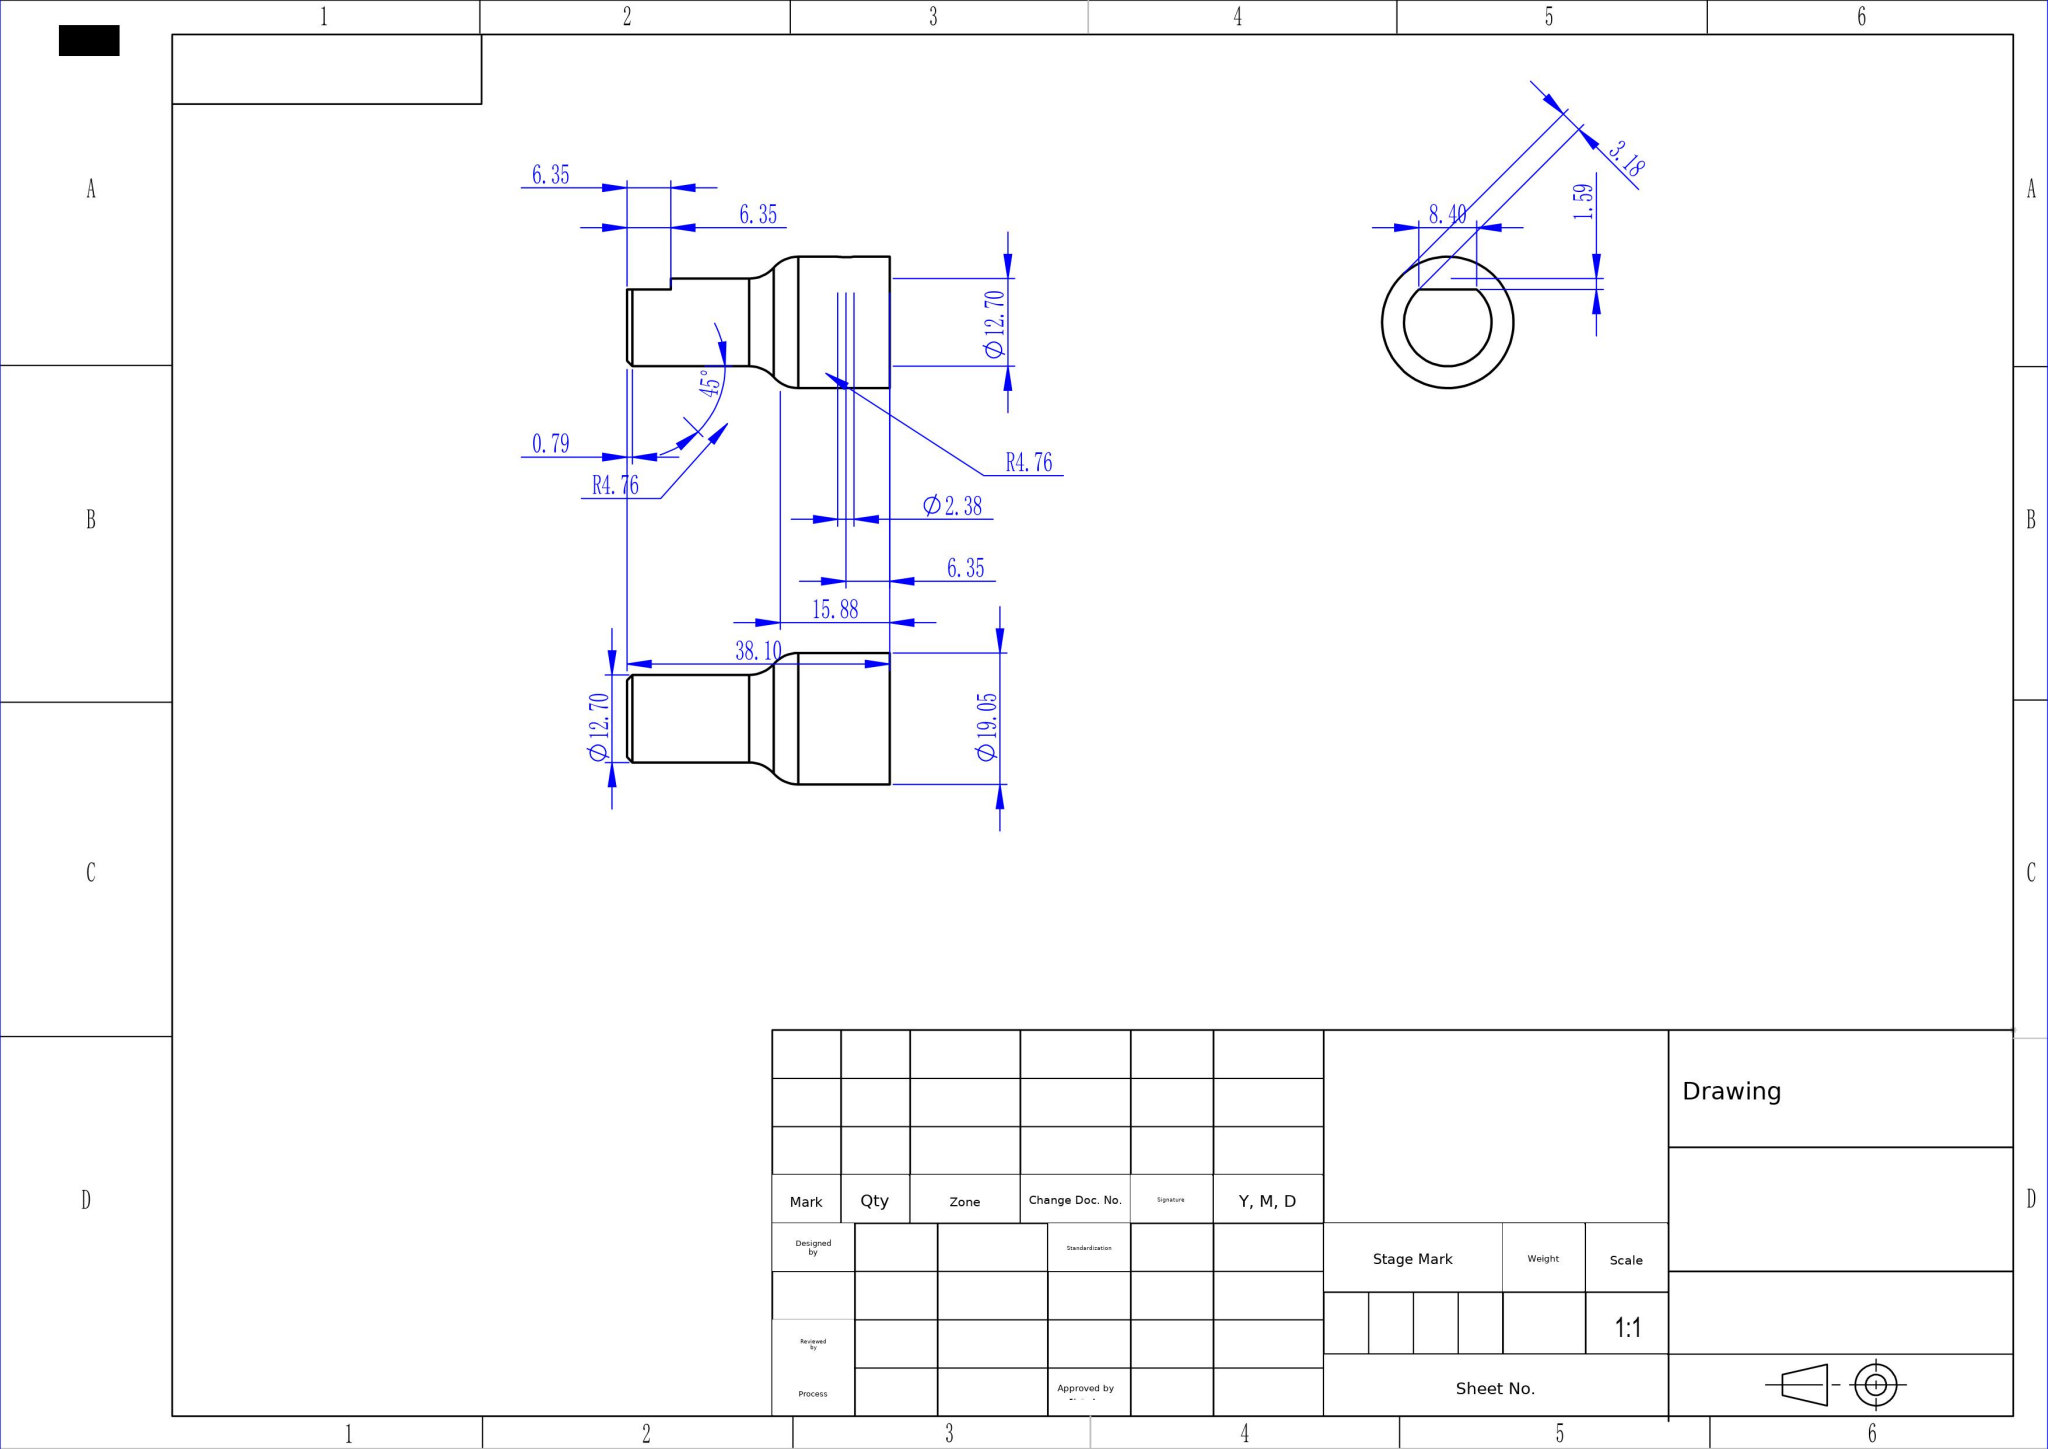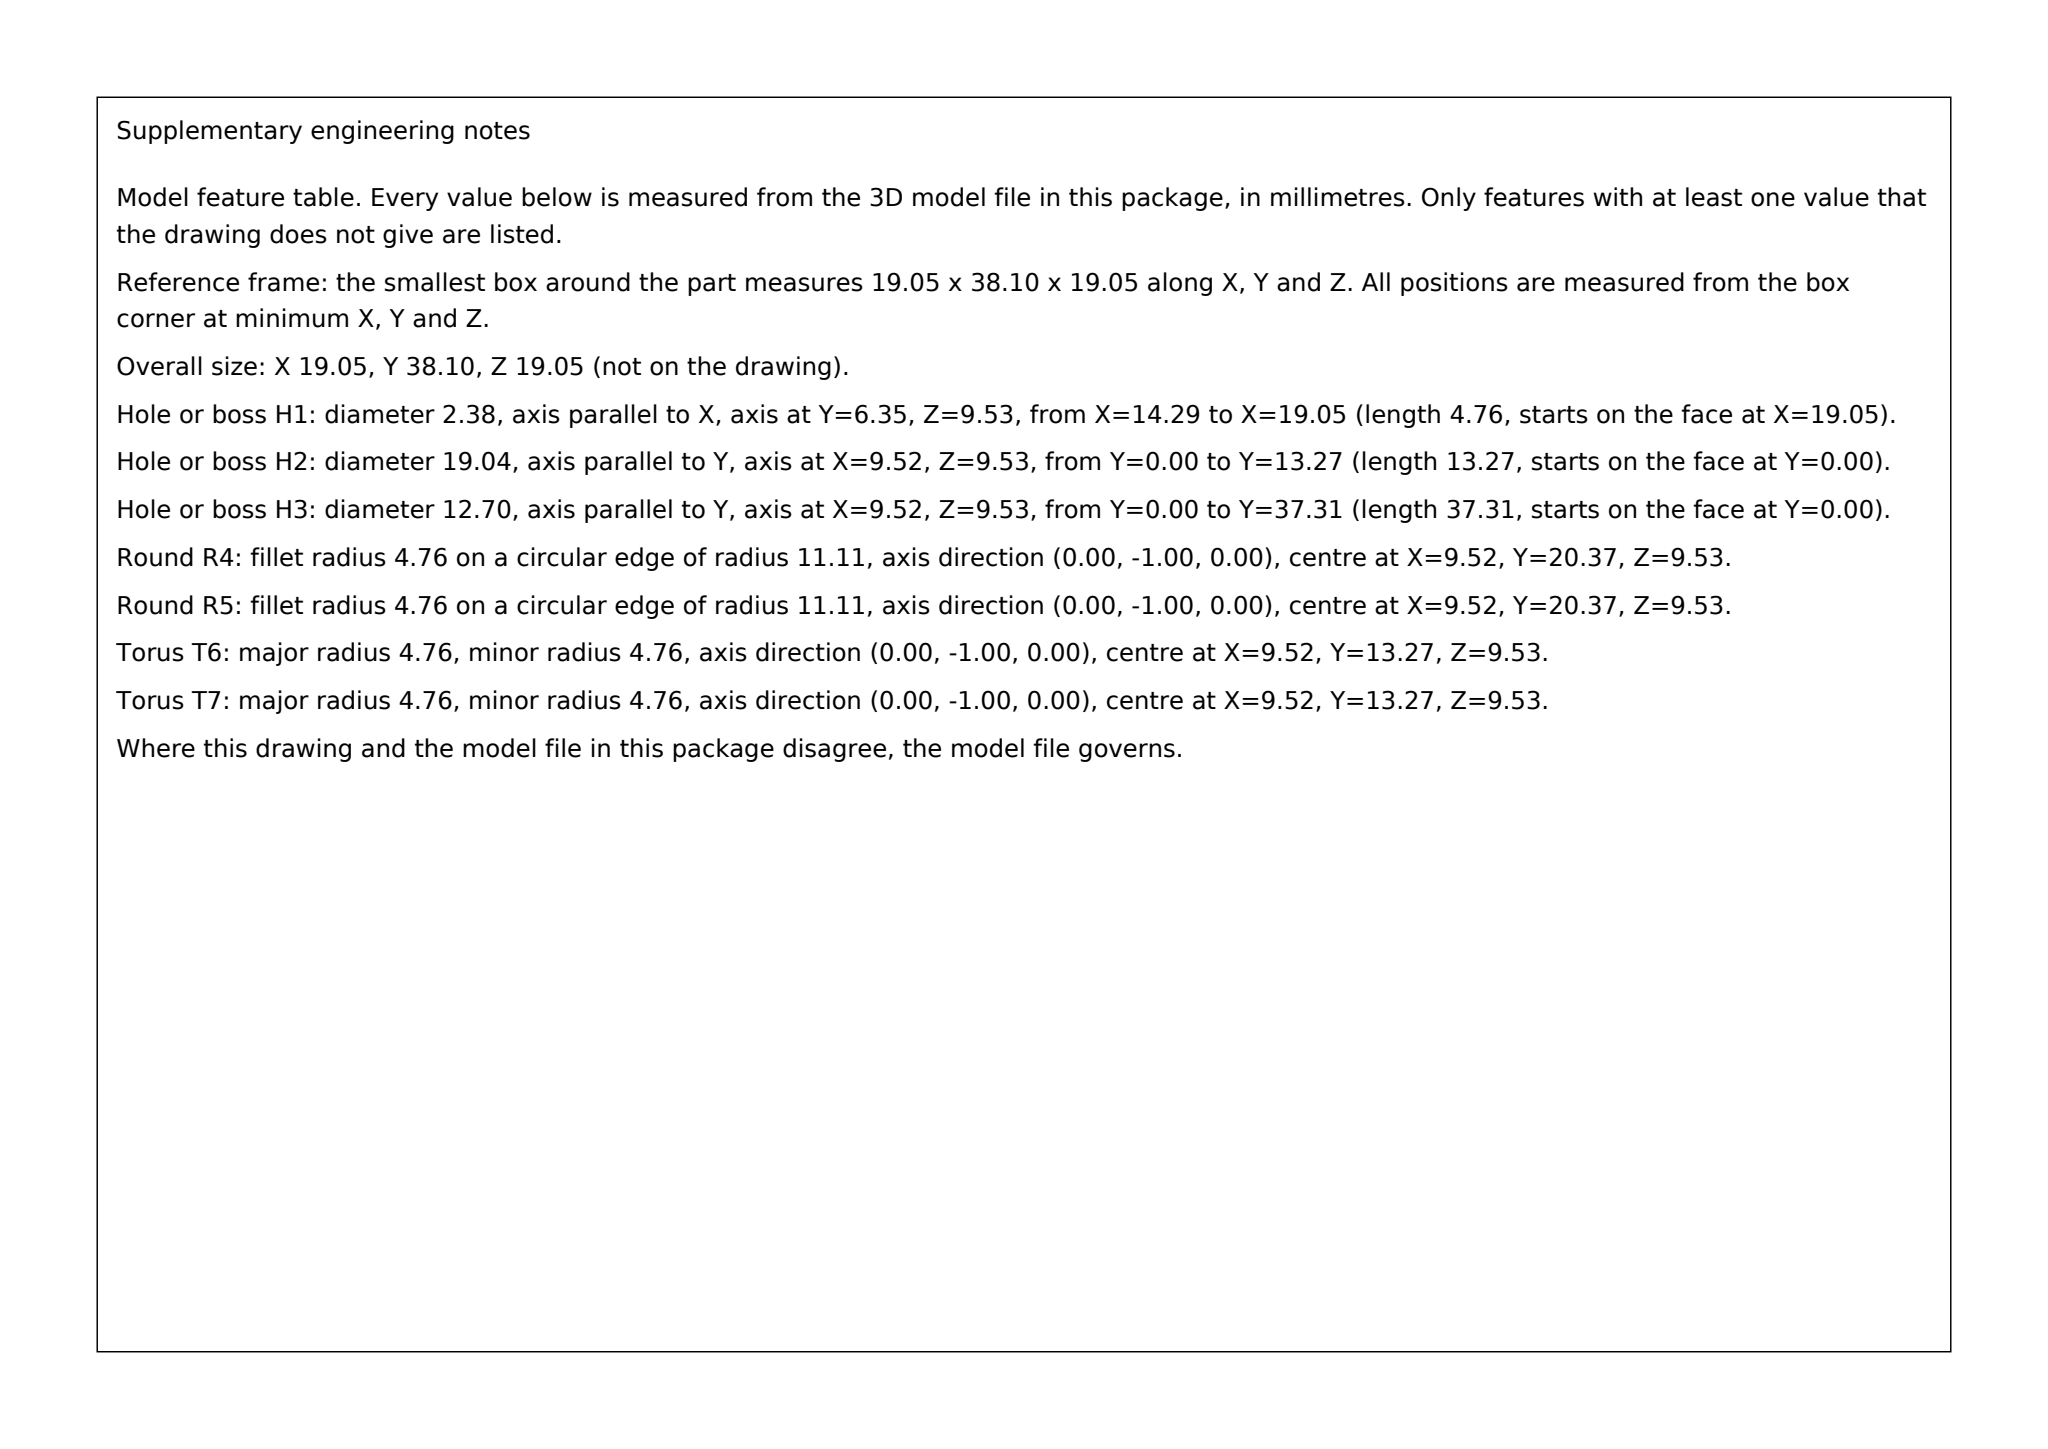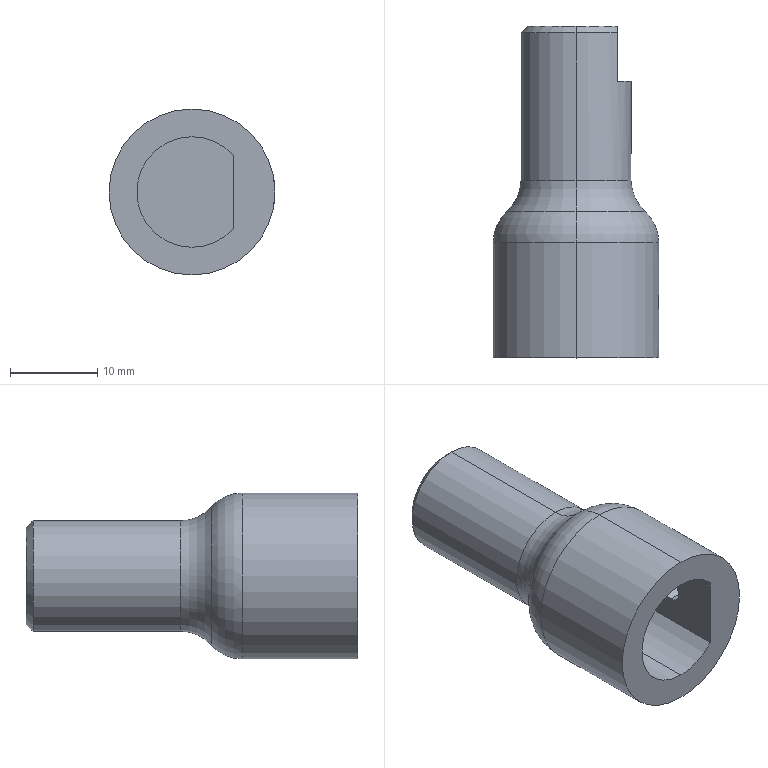Part | SolidWorks | drawing in inches | 1 solid | 22 faces | box 19.05 x 38.1 x 19.05 mm | volume 5883 mm3 | cylinder 9 | plane 6 | torus 4 | cone 3 | commonest cylinder face diameters 12.7 x5 2.381 x2 19.05 x2
STEP:
#1=CARTESIAN_POINT('',(0.,1.5,0.2187));
#2=VERTEX_POINT('',#1);
#3=CARTESIAN_POINT('',(0.1875,1.5,0.1127));
#4=VERTEX_POINT('',#3);
#5=CARTESIAN_POINT('',(0.,1.5,0.));
#6=DIRECTION('',(0.,1.,0.));
#7=DIRECTION('',(0.,0.,1.));
#8=AXIS2_PLACEMENT_3D('',#5,#6,#7);
#9=CIRCLE('',#8,0.2187);
#10=EDGE_CURVE('',#2,#4,#9,.T.);
#11=ORIENTED_EDGE('',*,*,#10,.F.);
#12=CARTESIAN_POINT('',(0.,1.469,0.25));
#13=VERTEX_POINT('',#12);
#14=CARTESIAN_POINT('',(0.,1.5,0.2187));
#15=DIRECTION('',(0.,-0.7071,0.7071));
#16=VECTOR('',#15,39.37);
#17=LINE('',#14,#16);
#18=EDGE_CURVE('',#2,#13,#17,.T.);
#19=ORIENTED_EDGE('',*,*,#18,.T.);
#20=CARTESIAN_POINT('',(0.1875,1.469,0.1654));
#21=VERTEX_POINT('',#20);
#22=CARTESIAN_POINT('',(0.,1.469,0.));
#23=DIRECTION('',(0.,-1.,0.));
#24=DIRECTION('',(0.,0.,1.));
#25=AXIS2_PLACEMENT_3D('',#22,#23,#24);
#26=CIRCLE('',#25,0.25);
#27=EDGE_CURVE('',#21,#13,#26,.T.);
#28=ORIENTED_EDGE('',*,*,#27,.F.);
#29=CARTESIAN_POINT('',(0.1875,1.5,0.1127));
#30=CARTESIAN_POINT('',(0.1875,1.491,0.1309));
#31=CARTESIAN_POINT('',(0.1875,1.48,0.1483));
#32=CARTESIAN_POINT('',(0.1875,1.469,0.1654));
#33=B_SPLINE_CURVE_WITH_KNOTS('',3,(#29,#30,#31,#32),.UNSPECIFIED.,.F.,.F.,(4,4),(0.,0.001556),.UNSPECIFIED.);
#34=EDGE_CURVE('',#4,#21,#33,.T.);
#35=ORIENTED_EDGE('',*,*,#34,.F.);
#36=EDGE_LOOP('',(#11,#19,#28,#35));
#37=FACE_OUTER_BOUND('',#36,.T.);
#38=CARTESIAN_POINT('',(0.,1.5,0.));
#39=DIRECTION('',(0.,-1.,0.));
#40=DIRECTION('',(0.,0.,-1.));
#41=AXIS2_PLACEMENT_3D('',#38,#39,#40);
#42=CONICAL_SURFACE('',#41,0.2187,0.7854);
#43=ADVANCED_FACE('',(#37),#42,.T.);
#44=ORIENTED_EDGE('',*,*,#18,.F.);
#45=CARTESIAN_POINT('',(0.,1.5,-0.2187));
#46=VERTEX_POINT('',#45);
#47=CARTESIAN_POINT('',(0.,1.5,0.));
#48=DIRECTION('',(0.,1.,0.));
#49=DIRECTION('',(0.,0.,1.));
#50=AXIS2_PLACEMENT_3D('',#47,#48,#49);
#51=CIRCLE('',#50,0.2187);
#52=EDGE_CURVE('',#46,#2,#51,.T.);
#53=ORIENTED_EDGE('',*,*,#52,.F.);
#54=CARTESIAN_POINT('',(0.,1.469,-0.25));
#55=VERTEX_POINT('',#54);
#56=CARTESIAN_POINT('',(0.,1.5,-0.2187));
#57=DIRECTION('',(0.,-0.7071,-0.7071));
#58=VECTOR('',#57,39.37);
#59=LINE('',#56,#58);
#60=EDGE_CURVE('',#46,#55,#59,.T.);
#61=ORIENTED_EDGE('',*,*,#60,.T.);
#62=CARTESIAN_POINT('',(0.,1.469,0.));
#63=DIRECTION('',(0.,-1.,0.));
#64=DIRECTION('',(0.,0.,1.));
#65=AXIS2_PLACEMENT_3D('',#62,#63,#64);
#66=CIRCLE('',#65,0.25);
#67=EDGE_CURVE('',#13,#55,#66,.T.);
#68=ORIENTED_EDGE('',*,*,#67,.F.);
#69=EDGE_LOOP('',(#44,#53,#61,#68));
#70=FACE_OUTER_BOUND('',#69,.T.);
#71=CARTESIAN_POINT('',(0.,1.5,0.));
#72=DIRECTION('',(0.,-1.,0.));
#73=DIRECTION('',(0.,0.,-1.));
#74=AXIS2_PLACEMENT_3D('',#71,#72,#73);
#75=CONICAL_SURFACE('',#74,0.2187,0.7854);
#76=ADVANCED_FACE('',(#70),#75,.T.);
#77=CARTESIAN_POINT('',(0.3721,0.25,-0.04687));
#78=VERTEX_POINT('',#77);
#79=CARTESIAN_POINT('',(0.3721,0.25,0.04688));
#80=VERTEX_POINT('',#79);
#81=CARTESIAN_POINT('',(0.3721,0.25,-0.04687));
#82=CARTESIAN_POINT('',(0.3721,0.2438,-0.04687));
#83=CARTESIAN_POINT('',(0.3722,0.2377,-0.04565));
#84=CARTESIAN_POINT('',(0.3728,0.2264,-0.04095));
#85=CARTESIAN_POINT('',(0.3731,0.2212,-0.03746));
#86=CARTESIAN_POINT('',(0.3739,0.2125,-0.02883));
#87=CARTESIAN_POINT('',(0.3743,0.209,-0.0236));
#88=CARTESIAN_POINT('',(0.3748,0.2044,-0.01233));
#89=CARTESIAN_POINT('',(0.375,0.2031,-0.006164));
#90=CARTESIAN_POINT('',(0.375,0.2031,0.006233));
#91=CARTESIAN_POINT('',(0.3748,0.2044,0.01232));
#92=CARTESIAN_POINT('',(0.3743,0.2091,0.02366));
#93=CARTESIAN_POINT('',(0.3739,0.2126,0.02885));
#94=CARTESIAN_POINT('',(0.3731,0.2212,0.03749));
#95=CARTESIAN_POINT('',(0.3728,0.2264,0.04097));
#96=CARTESIAN_POINT('',(0.3722,0.2377,0.04564));
#97=CARTESIAN_POINT('',(0.3721,0.2439,0.04688));
#98=CARTESIAN_POINT('',(0.3721,0.25,0.04688));
#99=B_SPLINE_CURVE_WITH_KNOTS('',3,(#81,#82,#83,#84,#85,#86,#87,#88,#89,#90,#91,#92,#93,#94,#95,#96,#97,#98),.UNSPECIFIED.,.F.,.F.,(4,2,2,2,2,2,2,2,4),(0.00559,0.006055,0.006521,0.006986,0.007452,0.007918,0.008383,0.008849,0.009315),.UNSPECIFIED.);
#100=EDGE_CURVE('',#78,#80,#99,.T.);
#101=ORIENTED_EDGE('',*,*,#100,.F.);
#102=CARTESIAN_POINT('',(0.1875,0.25,-0.04687));
#103=VERTEX_POINT('',#102);
#104=CARTESIAN_POINT('',(0.375,0.25,-0.04687));
#105=DIRECTION('',(-1.,0.,-0.));
#106=VECTOR('',#105,39.37);
#107=LINE('',#104,#106);
#108=EDGE_CURVE('',#78,#103,#107,.T.);
#109=ORIENTED_EDGE('',*,*,#108,.T.);
#110=CARTESIAN_POINT('',(0.1875,0.25,0.04688));
#111=VERTEX_POINT('',#110);
#112=CARTESIAN_POINT('',(0.1875,0.25,0.));
#113=DIRECTION('',(-1.,0.,-0.));
#114=DIRECTION('',(0.,0.,1.));
#115=AXIS2_PLACEMENT_3D('',#112,#113,#114);
#116=CIRCLE('',#115,0.04687);
#117=EDGE_CURVE('',#103,#111,#116,.T.);
#118=ORIENTED_EDGE('',*,*,#117,.T.);
#119=CARTESIAN_POINT('',(0.375,0.25,0.04688));
#120=DIRECTION('',(-1.,0.,-0.));
#121=VECTOR('',#120,39.37);
#122=LINE('',#119,#121);
#123=EDGE_CURVE('',#80,#111,#122,.T.);
#124=ORIENTED_EDGE('',*,*,#123,.F.);
#125=EDGE_LOOP('',(#101,#109,#118,#124));
#126=FACE_OUTER_BOUND('',#125,.T.);
#127=CARTESIAN_POINT('',(0.375,0.25,0.));
#128=DIRECTION('',(-1.,0.,-0.));
#129=DIRECTION('',(0.,0.,1.));
#130=AXIS2_PLACEMENT_3D('',#127,#128,#129);
#131=CYLINDRICAL_SURFACE('',#130,0.04687);
#132=ADVANCED_FACE('',(#126),#131,.F.);
#133=CARTESIAN_POINT('',(0.,0.662,0.3125));
#134=VERTEX_POINT('',#133);
#135=CARTESIAN_POINT('',(0.,0.662,-0.3125));
#136=VERTEX_POINT('',#135);
#137=CARTESIAN_POINT('',(0.,0.662,0.));
#138=DIRECTION('',(0.,1.,0.));
#139=DIRECTION('',(0.,0.,1.));
#140=AXIS2_PLACEMENT_3D('',#137,#138,#139);
#141=CIRCLE('',#140,0.3125);
#142=EDGE_CURVE('',#134,#136,#141,.T.);
#143=ORIENTED_EDGE('',*,*,#142,.F.);
#144=CARTESIAN_POINT('',(0.,0.5223,0.375));
#145=VERTEX_POINT('',#144);
#146=CARTESIAN_POINT('',(0.,0.5223,0.1875));
#147=DIRECTION('',(1.,0.,-0.));
#148=DIRECTION('',(-0.,0.,-1.));
#149=AXIS2_PLACEMENT_3D('',#146,#147,#148);
#150=CIRCLE('',#149,0.1875);
#151=EDGE_CURVE('',#134,#145,#150,.T.);
#152=ORIENTED_EDGE('',*,*,#151,.T.);
#153=CARTESIAN_POINT('',(0.,0.5223,-0.375));
#154=VERTEX_POINT('',#153);
#155=CARTESIAN_POINT('',(0.,0.5223,0.));
#156=DIRECTION('',(0.,-1.,0.));
#157=DIRECTION('',(0.,0.,-1.));
#158=AXIS2_PLACEMENT_3D('',#155,#156,#157);
#159=CIRCLE('',#158,0.375);
#160=EDGE_CURVE('',#154,#145,#159,.T.);
#161=ORIENTED_EDGE('',*,*,#160,.F.);
#162=CARTESIAN_POINT('',(0.,0.5223,-0.1875));
#163=DIRECTION('',(-1.,0.,0.));
#164=DIRECTION('',(0.,0.,1.));
#165=AXIS2_PLACEMENT_3D('',#162,#163,#164);
#166=CIRCLE('',#165,0.1875);
#167=EDGE_CURVE('',#136,#154,#166,.T.);
#168=ORIENTED_EDGE('',*,*,#167,.F.);
#169=EDGE_LOOP('',(#143,#152,#161,#168));
#170=FACE_OUTER_BOUND('',#169,.T.);
#171=CARTESIAN_POINT('',(0.,0.5223,0.));
#172=DIRECTION('',(0.,-1.,0.));
#173=DIRECTION('',(0.,0.,-1.));
#174=AXIS2_PLACEMENT_3D('',#171,#172,#173);
#175=TOROIDAL_SURFACE('',#174,0.1875,0.1875);
#176=ADVANCED_FACE('',(#170),#175,.T.);
#177=CARTESIAN_POINT('',(0.,0.662,0.));
#178=DIRECTION('',(0.,1.,0.));
#179=DIRECTION('',(0.,0.,1.));
#180=AXIS2_PLACEMENT_3D('',#177,#178,#179);
#181=CIRCLE('',#180,0.3125);
#182=EDGE_CURVE('',#136,#134,#181,.T.);
#183=ORIENTED_EDGE('',*,*,#182,.T.);
#184=CARTESIAN_POINT('',(0.,0.8018,0.25));
#185=VERTEX_POINT('',#184);
#186=CARTESIAN_POINT('',(0.,0.8018,0.4375));
#187=DIRECTION('',(1.,0.,-0.));
#188=DIRECTION('',(-0.,0.,-1.));
#189=AXIS2_PLACEMENT_3D('',#186,#187,#188);
#190=CIRCLE('',#189,0.1875);
#191=EDGE_CURVE('',#134,#185,#190,.T.);
#192=ORIENTED_EDGE('',*,*,#191,.T.);
#193=CARTESIAN_POINT('',(0.,0.8018,-0.25));
#194=VERTEX_POINT('',#193);
#195=CARTESIAN_POINT('',(0.,0.8018,0.));
#196=DIRECTION('',(0.,1.,0.));
#197=DIRECTION('',(0.,0.,-1.));
#198=AXIS2_PLACEMENT_3D('',#195,#196,#197);
#199=CIRCLE('',#198,0.25);
#200=EDGE_CURVE('',#194,#185,#199,.T.);
#201=ORIENTED_EDGE('',*,*,#200,.F.);
#202=CARTESIAN_POINT('',(0.,0.8018,-0.4375));
#203=DIRECTION('',(-1.,0.,0.));
#204=DIRECTION('',(0.,0.,1.));
#205=AXIS2_PLACEMENT_3D('',#202,#203,#204);
#206=CIRCLE('',#205,0.1875);
#207=EDGE_CURVE('',#136,#194,#206,.T.);
#208=ORIENTED_EDGE('',*,*,#207,.F.);
#209=EDGE_LOOP('',(#183,#192,#201,#208));
#210=FACE_OUTER_BOUND('',#209,.T.);
#211=CARTESIAN_POINT('',(0.,0.8018,0.));
#212=DIRECTION('',(0.,-1.,0.));
#213=DIRECTION('',(0.,0.,-1.));
#214=AXIS2_PLACEMENT_3D('',#211,#212,#213);
#215=TOROIDAL_SURFACE('',#214,0.4375,0.1875);
#216=ADVANCED_FACE('',(#210),#215,.F.);
#217=CARTESIAN_POINT('',(0.,0.5,-0.25));
#218=VERTEX_POINT('',#217);
#219=CARTESIAN_POINT('',(0.,0.5,0.25));
#220=VERTEX_POINT('',#219);
#221=CARTESIAN_POINT('',(0.,0.5,0.));
#222=DIRECTION('',(0.,1.,0.));
#223=DIRECTION('',(0.,0.,1.));
#224=AXIS2_PLACEMENT_3D('',#221,#222,#223);
#225=CIRCLE('',#224,0.25);
#226=EDGE_CURVE('',#218,#220,#225,.T.);
#227=ORIENTED_EDGE('',*,*,#226,.T.);
#228=CARTESIAN_POINT('',(0.,0.,0.25));
#229=VERTEX_POINT('',#228);
#230=CARTESIAN_POINT('',(0.,0.5,0.25));
#231=DIRECTION('',(0.,-1.,0.));
#232=VECTOR('',#231,39.37);
#233=LINE('',#230,#232);
#234=EDGE_CURVE('',#220,#229,#233,.T.);
#235=ORIENTED_EDGE('',*,*,#234,.T.);
#236=CARTESIAN_POINT('',(0.,0.,-0.25));
#237=VERTEX_POINT('',#236);
#238=CARTESIAN_POINT('',(0.,0.,0.));
#239=DIRECTION('',(0.,1.,0.));
#240=DIRECTION('',(0.,0.,1.));
#241=AXIS2_PLACEMENT_3D('',#238,#239,#240);
#242=CIRCLE('',#241,0.25);
#243=EDGE_CURVE('',#237,#229,#242,.T.);
#244=ORIENTED_EDGE('',*,*,#243,.F.);
#245=CARTESIAN_POINT('',(0.,0.5,-0.25));
#246=DIRECTION('',(0.,-1.,0.));
#247=VECTOR('',#246,39.37);
#248=LINE('',#245,#247);
#249=EDGE_CURVE('',#218,#237,#248,.T.);
#250=ORIENTED_EDGE('',*,*,#249,.F.);
#251=EDGE_LOOP('',(#227,#235,#244,#250));
#252=FACE_OUTER_BOUND('',#251,.T.);
#253=CARTESIAN_POINT('',(0.,0.5,0.));
#254=DIRECTION('',(0.,-1.,0.));
#255=DIRECTION('',(0.,0.,-1.));
#256=AXIS2_PLACEMENT_3D('',#253,#254,#255);
#257=CYLINDRICAL_SURFACE('',#256,0.25);
#258=ADVANCED_FACE('',(#252),#257,.F.);
#259=CARTESIAN_POINT('',(0.1875,0.5,-0.1654));
#260=VERTEX_POINT('',#259);
#261=CARTESIAN_POINT('',(0.,0.5,0.));
#262=DIRECTION('',(0.,1.,0.));
#263=DIRECTION('',(0.,0.,1.));
#264=AXIS2_PLACEMENT_3D('',#261,#262,#263);
#265=CIRCLE('',#264,0.25);
#266=EDGE_CURVE('',#260,#218,#265,.T.);
#267=ORIENTED_EDGE('',*,*,#266,.T.);
#268=ORIENTED_EDGE('',*,*,#249,.T.);
#269=CARTESIAN_POINT('',(0.1875,0.,-0.1654));
#270=VERTEX_POINT('',#269);
#271=CARTESIAN_POINT('',(0.,0.,0.));
#272=DIRECTION('',(0.,1.,0.));
#273=DIRECTION('',(0.,0.,1.));
#274=AXIS2_PLACEMENT_3D('',#271,#272,#273);
#275=CIRCLE('',#274,0.25);
#276=EDGE_CURVE('',#270,#237,#275,.T.);
#277=ORIENTED_EDGE('',*,*,#276,.F.);
#278=CARTESIAN_POINT('',(0.1875,0.5,-0.1654));
#279=DIRECTION('',(0.,-1.,0.));
#280=VECTOR('',#279,39.37);
#281=LINE('',#278,#280);
#282=EDGE_CURVE('',#260,#270,#281,.T.);
#283=ORIENTED_EDGE('',*,*,#282,.F.);
#284=EDGE_LOOP('',(#267,#268,#277,#283));
#285=FACE_OUTER_BOUND('',#284,.T.);
#286=CARTESIAN_POINT('',(0.,0.5,0.));
#287=DIRECTION('',(0.,-1.,0.));
#288=DIRECTION('',(0.,0.,-1.));
#289=AXIS2_PLACEMENT_3D('',#286,#287,#288);
#290=CYLINDRICAL_SURFACE('',#289,0.25);
#291=ADVANCED_FACE('',(#285),#290,.F.);
#292=CARTESIAN_POINT('',(0.3721,0.25,0.04688));
#293=CARTESIAN_POINT('',(0.3721,0.2561,0.04688));
#294=CARTESIAN_POINT('',(0.3722,0.2623,0.04566));
#295=CARTESIAN_POINT('',(0.3728,0.2736,0.04095));
#296=CARTESIAN_POINT('',(0.3731,0.2788,0.03751));
#297=CARTESIAN_POINT('',(0.3739,0.2875,0.02876));
#298=CARTESIAN_POINT('',(0.3743,0.291,0.0236));
#299=CARTESIAN_POINT('',(0.3748,0.2957,0.01225));
#300=CARTESIAN_POINT('',(0.375,0.2969,0.006105));
#301=CARTESIAN_POINT('',(0.375,0.2969,-0.006138));
#302=CARTESIAN_POINT('',(0.3748,0.2956,-0.01231));
#303=CARTESIAN_POINT('',(0.3743,0.291,-0.02359));
#304=CARTESIAN_POINT('',(0.3739,0.2875,-0.02882));
#305=CARTESIAN_POINT('',(0.3731,0.2788,-0.03746));
#306=CARTESIAN_POINT('',(0.3728,0.2736,-0.04094));
#307=CARTESIAN_POINT('',(0.3722,0.2623,-0.04565));
#308=CARTESIAN_POINT('',(0.3721,0.2562,-0.04687));
#309=CARTESIAN_POINT('',(0.3721,0.25,-0.04687));
#310=B_SPLINE_CURVE_WITH_KNOTS('',3,(#292,#293,#294,#295,#296,#297,#298,#299,#300,#301,#302,#303,#304,#305,#306,#307,#308,#309),.UNSPECIFIED.,.F.,.F.,(4,2,2,2,2,2,2,2,4),(0.001863,0.002329,0.002795,0.003261,0.003726,0.004192,0.004658,0.005124,0.00559),.UNSPECIFIED.);
#311=EDGE_CURVE('',#80,#78,#310,.T.);
#312=ORIENTED_EDGE('',*,*,#311,.T.);
#313=ORIENTED_EDGE('',*,*,#100,.T.);
#314=EDGE_LOOP('',(#312,#313));
#315=FACE_BOUND('',#314,.T.);
#316=ORIENTED_EDGE('',*,*,#160,.T.);
#317=CARTESIAN_POINT('',(0.,0.,0.375));
#318=VERTEX_POINT('',#317);
#319=CARTESIAN_POINT('',(0.,0.625,0.375));
#320=DIRECTION('',(0.,-1.,0.));
#321=VECTOR('',#320,39.37);
#322=LINE('',#319,#321);
#323=EDGE_CURVE('',#145,#318,#322,.T.);
#324=ORIENTED_EDGE('',*,*,#323,.T.);
#325=CARTESIAN_POINT('',(0.,0.,-0.375));
#326=VERTEX_POINT('',#325);
#327=CARTESIAN_POINT('',(0.,0.,0.));
#328=DIRECTION('',(0.,1.,0.));
#329=DIRECTION('',(0.,0.,1.));
#330=AXIS2_PLACEMENT_3D('',#327,#328,#329);
#331=CIRCLE('',#330,0.375);
#332=EDGE_CURVE('',#318,#326,#331,.T.);
#333=ORIENTED_EDGE('',*,*,#332,.T.);
#334=CARTESIAN_POINT('',(0.,0.625,-0.375));
#335=DIRECTION('',(0.,-1.,0.));
#336=VECTOR('',#335,39.37);
#337=LINE('',#334,#336);
#338=EDGE_CURVE('',#154,#326,#337,.T.);
#339=ORIENTED_EDGE('',*,*,#338,.F.);
#340=EDGE_LOOP('',(#316,#324,#333,#339));
#341=FACE_OUTER_BOUND('',#340,.T.);
#342=CARTESIAN_POINT('',(0.,0.625,0.));
#343=DIRECTION('',(0.,-1.,0.));
#344=DIRECTION('',(0.,0.,-1.));
#345=AXIS2_PLACEMENT_3D('',#342,#343,#344);
#346=CYLINDRICAL_SURFACE('',#345,0.375);
#347=ADVANCED_FACE('',(#315,#341),#346,.T.);
#348=ORIENTED_EDGE('',*,*,#27,.T.);
#349=CARTESIAN_POINT('',(0.,1.5,0.25));
#350=DIRECTION('',(0.,-1.,0.));
#351=VECTOR('',#350,39.37);
#352=LINE('',#349,#351);
#353=EDGE_CURVE('',#13,#185,#352,.T.);
#354=ORIENTED_EDGE('',*,*,#353,.T.);
#355=CARTESIAN_POINT('',(0.,0.8018,0.));
#356=DIRECTION('',(0.,1.,0.));
#357=DIRECTION('',(0.,0.,-1.));
#358=AXIS2_PLACEMENT_3D('',#355,#356,#357);
#359=CIRCLE('',#358,0.25);
#360=EDGE_CURVE('',#185,#194,#359,.T.);
#361=ORIENTED_EDGE('',*,*,#360,.T.);
#362=CARTESIAN_POINT('',(0.,1.5,-0.25));
#363=DIRECTION('',(0.,-1.,0.));
#364=VECTOR('',#363,39.37);
#365=LINE('',#362,#364);
#366=EDGE_CURVE('',#55,#194,#365,.T.);
#367=ORIENTED_EDGE('',*,*,#366,.F.);
#368=CARTESIAN_POINT('',(0.1875,1.469,-0.1654));
#369=VERTEX_POINT('',#368);
#370=CARTESIAN_POINT('',(0.,1.469,0.));
#371=DIRECTION('',(0.,-1.,0.));
#372=DIRECTION('',(0.,0.,1.));
#373=AXIS2_PLACEMENT_3D('',#370,#371,#372);
#374=CIRCLE('',#373,0.25);
#375=EDGE_CURVE('',#55,#369,#374,.T.);
#376=ORIENTED_EDGE('',*,*,#375,.T.);
#377=CARTESIAN_POINT('',(0.1875,1.25,-0.1654));
#378=VERTEX_POINT('',#377);
#379=CARTESIAN_POINT('',(0.1875,1.25,-0.1654));
#380=DIRECTION('',(0.,1.,0.));
#381=VECTOR('',#380,39.37);
#382=LINE('',#379,#381);
#383=EDGE_CURVE('',#378,#369,#382,.T.);
#384=ORIENTED_EDGE('',*,*,#383,.F.);
#385=CARTESIAN_POINT('',(0.1875,1.25,0.1654));
#386=VERTEX_POINT('',#385);
#387=CARTESIAN_POINT('',(0.,1.25,0.));
#388=DIRECTION('',(0.,1.,0.));
#389=DIRECTION('',(0.,0.,1.));
#390=AXIS2_PLACEMENT_3D('',#387,#388,#389);
#391=CIRCLE('',#390,0.25);
#392=EDGE_CURVE('',#386,#378,#391,.T.);
#393=ORIENTED_EDGE('',*,*,#392,.F.);
#394=CARTESIAN_POINT('',(0.1875,1.25,0.1654));
#395=DIRECTION('',(0.,1.,0.));
#396=VECTOR('',#395,39.37);
#397=LINE('',#394,#396);
#398=EDGE_CURVE('',#386,#21,#397,.T.);
#399=ORIENTED_EDGE('',*,*,#398,.T.);
#400=EDGE_LOOP('',(#348,#354,#361,#367,#376,#384,#393,#399));
#401=FACE_OUTER_BOUND('',#400,.T.);
#402=CARTESIAN_POINT('',(0.,1.5,0.));
#403=DIRECTION('',(0.,-1.,0.));
#404=DIRECTION('',(0.,0.,-1.));
#405=AXIS2_PLACEMENT_3D('',#402,#403,#404);
#406=CYLINDRICAL_SURFACE('',#405,0.25);
#407=ADVANCED_FACE('',(#401),#406,.T.);
#408=ORIENTED_EDGE('',*,*,#353,.F.);
#409=ORIENTED_EDGE('',*,*,#67,.T.);
#410=ORIENTED_EDGE('',*,*,#366,.T.);
#411=ORIENTED_EDGE('',*,*,#200,.T.);
#412=EDGE_LOOP('',(#408,#409,#410,#411));
#413=FACE_OUTER_BOUND('',#412,.T.);
#414=CARTESIAN_POINT('',(0.,1.5,0.));
#415=DIRECTION('',(0.,-1.,0.));
#416=DIRECTION('',(0.,0.,-1.));
#417=AXIS2_PLACEMENT_3D('',#414,#415,#416);
#418=CYLINDRICAL_SURFACE('',#417,0.25);
#419=ADVANCED_FACE('',(#413),#418,.T.);
#420=CARTESIAN_POINT('',(0.1875,1.5,-0.1127));
#421=VERTEX_POINT('',#420);
#422=CARTESIAN_POINT('',(0.1875,1.5,0.1654));
#423=DIRECTION('',(0.,0.,-1.));
#424=VECTOR('',#423,39.37);
#425=LINE('',#422,#424);
#426=EDGE_CURVE('',#4,#421,#425,.T.);
#427=ORIENTED_EDGE('',*,*,#426,.T.);
#428=CARTESIAN_POINT('',(0.,1.5,0.));
#429=DIRECTION('',(0.,1.,0.));
#430=DIRECTION('',(0.,0.,1.));
#431=AXIS2_PLACEMENT_3D('',#428,#429,#430);
#432=CIRCLE('',#431,0.2187);
#433=EDGE_CURVE('',#421,#46,#432,.T.);
#434=ORIENTED_EDGE('',*,*,#433,.T.);
#435=ORIENTED_EDGE('',*,*,#52,.T.);
#436=ORIENTED_EDGE('',*,*,#10,.T.);
#437=EDGE_LOOP('',(#427,#434,#435,#436));
#438=FACE_OUTER_BOUND('',#437,.T.);
#439=CARTESIAN_POINT('',(0.,1.5,0.));
#440=DIRECTION('',(0.,1.,0.));
#441=DIRECTION('',(0.,0.,1.));
#442=AXIS2_PLACEMENT_3D('',#439,#440,#441);
#443=PLANE('',#442);
#444=ADVANCED_FACE('',(#438),#443,.T.);
#445=CARTESIAN_POINT('',(0.,0.,0.));
#446=DIRECTION('',(0.,1.,0.));
#447=DIRECTION('',(0.,0.,1.));
#448=AXIS2_PLACEMENT_3D('',#445,#446,#447);
#449=CIRCLE('',#448,0.375);
#450=EDGE_CURVE('',#326,#318,#449,.T.);
#451=ORIENTED_EDGE('',*,*,#450,.F.);
#452=ORIENTED_EDGE('',*,*,#332,.F.);
#453=EDGE_LOOP('',(#451,#452));
#454=FACE_OUTER_BOUND('',#453,.T.);
#455=ORIENTED_EDGE('',*,*,#276,.T.);
#456=ORIENTED_EDGE('',*,*,#243,.T.);
#457=CARTESIAN_POINT('',(0.1875,0.,0.1654));
#458=VERTEX_POINT('',#457);
#459=CARTESIAN_POINT('',(0.,0.,0.));
#460=DIRECTION('',(0.,1.,0.));
#461=DIRECTION('',(0.,0.,1.));
#462=AXIS2_PLACEMENT_3D('',#459,#460,#461);
#463=CIRCLE('',#462,0.25);
#464=EDGE_CURVE('',#229,#458,#463,.T.);
#465=ORIENTED_EDGE('',*,*,#464,.T.);
#466=CARTESIAN_POINT('',(0.1875,0.,0.1654));
#467=DIRECTION('',(0.,0.,-1.));
#468=VECTOR('',#467,39.37);
#469=LINE('',#466,#468);
#470=EDGE_CURVE('',#458,#270,#469,.T.);
#471=ORIENTED_EDGE('',*,*,#470,.T.);
#472=EDGE_LOOP('',(#455,#456,#465,#471));
#473=FACE_BOUND('',#472,.T.);
#474=CARTESIAN_POINT('',(0.,0.,0.));
#475=DIRECTION('',(0.,1.,0.));
#476=DIRECTION('',(0.,0.,1.));
#477=AXIS2_PLACEMENT_3D('',#474,#475,#476);
#478=PLANE('',#477);
#479=ADVANCED_FACE('',(#454,#473),#478,.F.);
#480=ORIENTED_EDGE('',*,*,#323,.F.);
#481=CARTESIAN_POINT('',(0.,0.5223,0.));
#482=DIRECTION('',(0.,-1.,0.));
#483=DIRECTION('',(0.,0.,-1.));
#484=AXIS2_PLACEMENT_3D('',#481,#482,#483);
#485=CIRCLE('',#484,0.375);
#486=EDGE_CURVE('',#145,#154,#485,.T.);
#487=ORIENTED_EDGE('',*,*,#486,.T.);
#488=ORIENTED_EDGE('',*,*,#338,.T.);
#489=ORIENTED_EDGE('',*,*,#450,.T.);
#490=EDGE_LOOP('',(#480,#487,#488,#489));
#491=FACE_OUTER_BOUND('',#490,.T.);
#492=CARTESIAN_POINT('',(0.,0.625,0.));
#493=DIRECTION('',(0.,-1.,0.));
#494=DIRECTION('',(0.,0.,-1.));
#495=AXIS2_PLACEMENT_3D('',#492,#493,#494);
#496=CYLINDRICAL_SURFACE('',#495,0.375);
#497=ADVANCED_FACE('',(#491),#496,.T.);
#498=ORIENTED_EDGE('',*,*,#234,.F.);
#499=CARTESIAN_POINT('',(0.1875,0.5,0.1654));
#500=VERTEX_POINT('',#499);
#501=CARTESIAN_POINT('',(0.,0.5,0.));
#502=DIRECTION('',(0.,1.,0.));
#503=DIRECTION('',(0.,0.,1.));
#504=AXIS2_PLACEMENT_3D('',#501,#502,#503);
#505=CIRCLE('',#504,0.25);
#506=EDGE_CURVE('',#220,#500,#505,.T.);
#507=ORIENTED_EDGE('',*,*,#506,.T.);
#508=CARTESIAN_POINT('',(0.1875,0.5,0.1654));
#509=DIRECTION('',(0.,-1.,0.));
#510=VECTOR('',#509,39.37);
#511=LINE('',#508,#510);
#512=EDGE_CURVE('',#500,#458,#511,.T.);
#513=ORIENTED_EDGE('',*,*,#512,.T.);
#514=ORIENTED_EDGE('',*,*,#464,.F.);
#515=EDGE_LOOP('',(#498,#507,#513,#514));
#516=FACE_OUTER_BOUND('',#515,.T.);
#517=CARTESIAN_POINT('',(0.,0.5,0.));
#518=DIRECTION('',(0.,-1.,0.));
#519=DIRECTION('',(0.,0.,-1.));
#520=AXIS2_PLACEMENT_3D('',#517,#518,#519);
#521=CYLINDRICAL_SURFACE('',#520,0.25);
#522=ADVANCED_FACE('',(#516),#521,.F.);
#523=CARTESIAN_POINT('',(0.1875,0.25,0.));
#524=DIRECTION('',(-1.,0.,-0.));
#525=DIRECTION('',(0.,0.,1.));
#526=AXIS2_PLACEMENT_3D('',#523,#524,#525);
#527=CIRCLE('',#526,0.04687);
#528=EDGE_CURVE('',#111,#103,#527,.T.);
#529=ORIENTED_EDGE('',*,*,#528,.F.);
#530=ORIENTED_EDGE('',*,*,#117,.F.);
#531=EDGE_LOOP('',(#529,#530));
#532=FACE_BOUND('',#531,.T.);
#533=ORIENTED_EDGE('',*,*,#470,.F.);
#534=ORIENTED_EDGE('',*,*,#512,.F.);
#535=CARTESIAN_POINT('',(0.1875,0.5,0.1654));
#536=DIRECTION('',(0.,0.,-1.));
#537=VECTOR('',#536,39.37);
#538=LINE('',#535,#537);
#539=EDGE_CURVE('',#500,#260,#538,.T.);
#540=ORIENTED_EDGE('',*,*,#539,.T.);
#541=ORIENTED_EDGE('',*,*,#282,.T.);
#542=EDGE_LOOP('',(#533,#534,#540,#541));
#543=FACE_OUTER_BOUND('',#542,.T.);
#544=CARTESIAN_POINT('',(0.1875,0.5,0.1654));
#545=DIRECTION('',(-1.,0.,-0.));
#546=DIRECTION('',(-0.,0.,1.));
#547=AXIS2_PLACEMENT_3D('',#544,#545,#546);
#548=PLANE('',#547);
#549=ADVANCED_FACE('',(#532,#543),#548,.T.);
#550=ORIENTED_EDGE('',*,*,#266,.F.);
#551=ORIENTED_EDGE('',*,*,#539,.F.);
#552=ORIENTED_EDGE('',*,*,#506,.F.);
#553=ORIENTED_EDGE('',*,*,#226,.F.);
#554=EDGE_LOOP('',(#550,#551,#552,#553));
#555=FACE_OUTER_BOUND('',#554,.T.);
#556=CARTESIAN_POINT('',(0.,0.5,0.));
#557=DIRECTION('',(0.,1.,0.));
#558=DIRECTION('',(0.,0.,1.));
#559=AXIS2_PLACEMENT_3D('',#556,#557,#558);
#560=PLANE('',#559);
#561=ADVANCED_FACE('',(#555),#560,.F.);
#562=ORIENTED_EDGE('',*,*,#191,.F.);
#563=ORIENTED_EDGE('',*,*,#142,.T.);
#564=ORIENTED_EDGE('',*,*,#207,.T.);
#565=ORIENTED_EDGE('',*,*,#360,.F.);
#566=EDGE_LOOP('',(#562,#563,#564,#565));
#567=FACE_OUTER_BOUND('',#566,.T.);
#568=CARTESIAN_POINT('',(0.,0.8018,0.));
#569=DIRECTION('',(0.,-1.,0.));
#570=DIRECTION('',(0.,0.,-1.));
#571=AXIS2_PLACEMENT_3D('',#568,#569,#570);
#572=TOROIDAL_SURFACE('',#571,0.4375,0.1875);
#573=ADVANCED_FACE('',(#567),#572,.F.);
#574=ORIENTED_EDGE('',*,*,#151,.F.);
#575=ORIENTED_EDGE('',*,*,#182,.F.);
#576=ORIENTED_EDGE('',*,*,#167,.T.);
#577=ORIENTED_EDGE('',*,*,#486,.F.);
#578=EDGE_LOOP('',(#574,#575,#576,#577));
#579=FACE_OUTER_BOUND('',#578,.T.);
#580=CARTESIAN_POINT('',(0.,0.5223,0.));
#581=DIRECTION('',(0.,-1.,0.));
#582=DIRECTION('',(0.,0.,-1.));
#583=AXIS2_PLACEMENT_3D('',#580,#581,#582);
#584=TOROIDAL_SURFACE('',#583,0.1875,0.1875);
#585=ADVANCED_FACE('',(#579),#584,.T.);
#586=ORIENTED_EDGE('',*,*,#108,.F.);
#587=ORIENTED_EDGE('',*,*,#311,.F.);
#588=ORIENTED_EDGE('',*,*,#123,.T.);
#589=ORIENTED_EDGE('',*,*,#528,.T.);
#590=EDGE_LOOP('',(#586,#587,#588,#589));
#591=FACE_OUTER_BOUND('',#590,.T.);
#592=CARTESIAN_POINT('',(0.375,0.25,0.));
#593=DIRECTION('',(-1.,0.,-0.));
#594=DIRECTION('',(0.,0.,1.));
#595=AXIS2_PLACEMENT_3D('',#592,#593,#594);
#596=CYLINDRICAL_SURFACE('',#595,0.04687);
#597=ADVANCED_FACE('',(#591),#596,.F.);
#598=ORIENTED_EDGE('',*,*,#426,.F.);
#599=ORIENTED_EDGE('',*,*,#34,.T.);
#600=ORIENTED_EDGE('',*,*,#398,.F.);
#601=CARTESIAN_POINT('',(0.1875,1.25,0.1654));
#602=DIRECTION('',(0.,0.,-1.));
#603=VECTOR('',#602,39.37);
#604=LINE('',#601,#603);
#605=EDGE_CURVE('',#386,#378,#604,.T.);
#606=ORIENTED_EDGE('',*,*,#605,.T.);
#607=ORIENTED_EDGE('',*,*,#383,.T.);
#608=CARTESIAN_POINT('',(0.1875,1.469,-0.1654));
#609=CARTESIAN_POINT('',(0.1875,1.48,-0.1483));
#610=CARTESIAN_POINT('',(0.1875,1.491,-0.1309));
#611=CARTESIAN_POINT('',(0.1875,1.5,-0.1127));
#612=B_SPLINE_CURVE_WITH_KNOTS('',3,(#608,#609,#610,#611),.UNSPECIFIED.,.F.,.F.,(4,4),(0.,0.001556),.UNSPECIFIED.);
#613=EDGE_CURVE('',#369,#421,#612,.T.);
#614=ORIENTED_EDGE('',*,*,#613,.T.);
#615=EDGE_LOOP('',(#598,#599,#600,#606,#607,#614));
#616=FACE_OUTER_BOUND('',#615,.T.);
#617=CARTESIAN_POINT('',(0.1875,1.25,0.1654));
#618=DIRECTION('',(1.,0.,0.));
#619=DIRECTION('',(0.,0.,-1.));
#620=AXIS2_PLACEMENT_3D('',#617,#618,#619);
#621=PLANE('',#620);
#622=ADVANCED_FACE('',(#616),#621,.T.);
#623=ORIENTED_EDGE('',*,*,#392,.T.);
#624=ORIENTED_EDGE('',*,*,#605,.F.);
#625=EDGE_LOOP('',(#623,#624));
#626=FACE_OUTER_BOUND('',#625,.T.);
#627=CARTESIAN_POINT('',(0.,1.25,0.));
#628=DIRECTION('',(0.,1.,0.));
#629=DIRECTION('',(0.,0.,1.));
#630=AXIS2_PLACEMENT_3D('',#627,#628,#629);
#631=PLANE('',#630);
#632=ADVANCED_FACE('',(#626),#631,.T.);
#633=ORIENTED_EDGE('',*,*,#60,.F.);
#634=ORIENTED_EDGE('',*,*,#433,.F.);
#635=ORIENTED_EDGE('',*,*,#613,.F.);
#636=ORIENTED_EDGE('',*,*,#375,.F.);
#637=EDGE_LOOP('',(#633,#634,#635,#636));
#638=FACE_OUTER_BOUND('',#637,.T.);
#639=CARTESIAN_POINT('',(0.,1.5,0.));
#640=DIRECTION('',(0.,-1.,0.));
#641=DIRECTION('',(0.,0.,-1.));
#642=AXIS2_PLACEMENT_3D('',#639,#640,#641);
#643=CONICAL_SURFACE('',#642,0.2187,0.7854);
#644=ADVANCED_FACE('',(#638),#643,.T.);
#645=CLOSED_SHELL('',(#43,#76,#132,#176,#216,#258,#291,#347,#407,#419,#444,#479,#497,#522,#549,#561,#573,#585,#597,#622,#632,#644));
#646=MANIFOLD_SOLID_BREP('',#645);
#647=CARTESIAN_POINT('',(0.,0.,0.));
#648=DIRECTION('',(0.,0.,1.));
#649=DIRECTION('',(1.,0.,0.));
#650=AXIS2_PLACEMENT_3D('',#647,#648,#649);
#651=(LENGTH_UNIT()NAMED_UNIT(*)SI_UNIT($,.METRE.));
#652=LENGTH_MEASURE_WITH_UNIT(LENGTH_MEASURE(0.0254),#651);
#653=DIMENSIONAL_EXPONENTS(1.,0.,0.,0.,0.,0.,0.);
#654=(CONVERSION_BASED_UNIT('',#652)LENGTH_UNIT()NAMED_UNIT(#653));
#655=UNCERTAINTY_MEASURE_WITH_UNIT(LENGTH_MEASURE(0.00001),#654,'','');
#656=(NAMED_UNIT(*)PLANE_ANGLE_UNIT()SI_UNIT($,.RADIAN.));
#657=(NAMED_UNIT(*)SI_UNIT($,.STERADIAN.)SOLID_ANGLE_UNIT());
#658=(GEOMETRIC_REPRESENTATION_CONTEXT(3)GLOBAL_UNCERTAINTY_ASSIGNED_CONTEXT((#655))GLOBAL_UNIT_ASSIGNED_CONTEXT((#654,#656,#657))REPRESENTATION_CONTEXT('',''));
#659=ADVANCED_BREP_SHAPE_REPRESENTATION('',(#646,#650),#658);